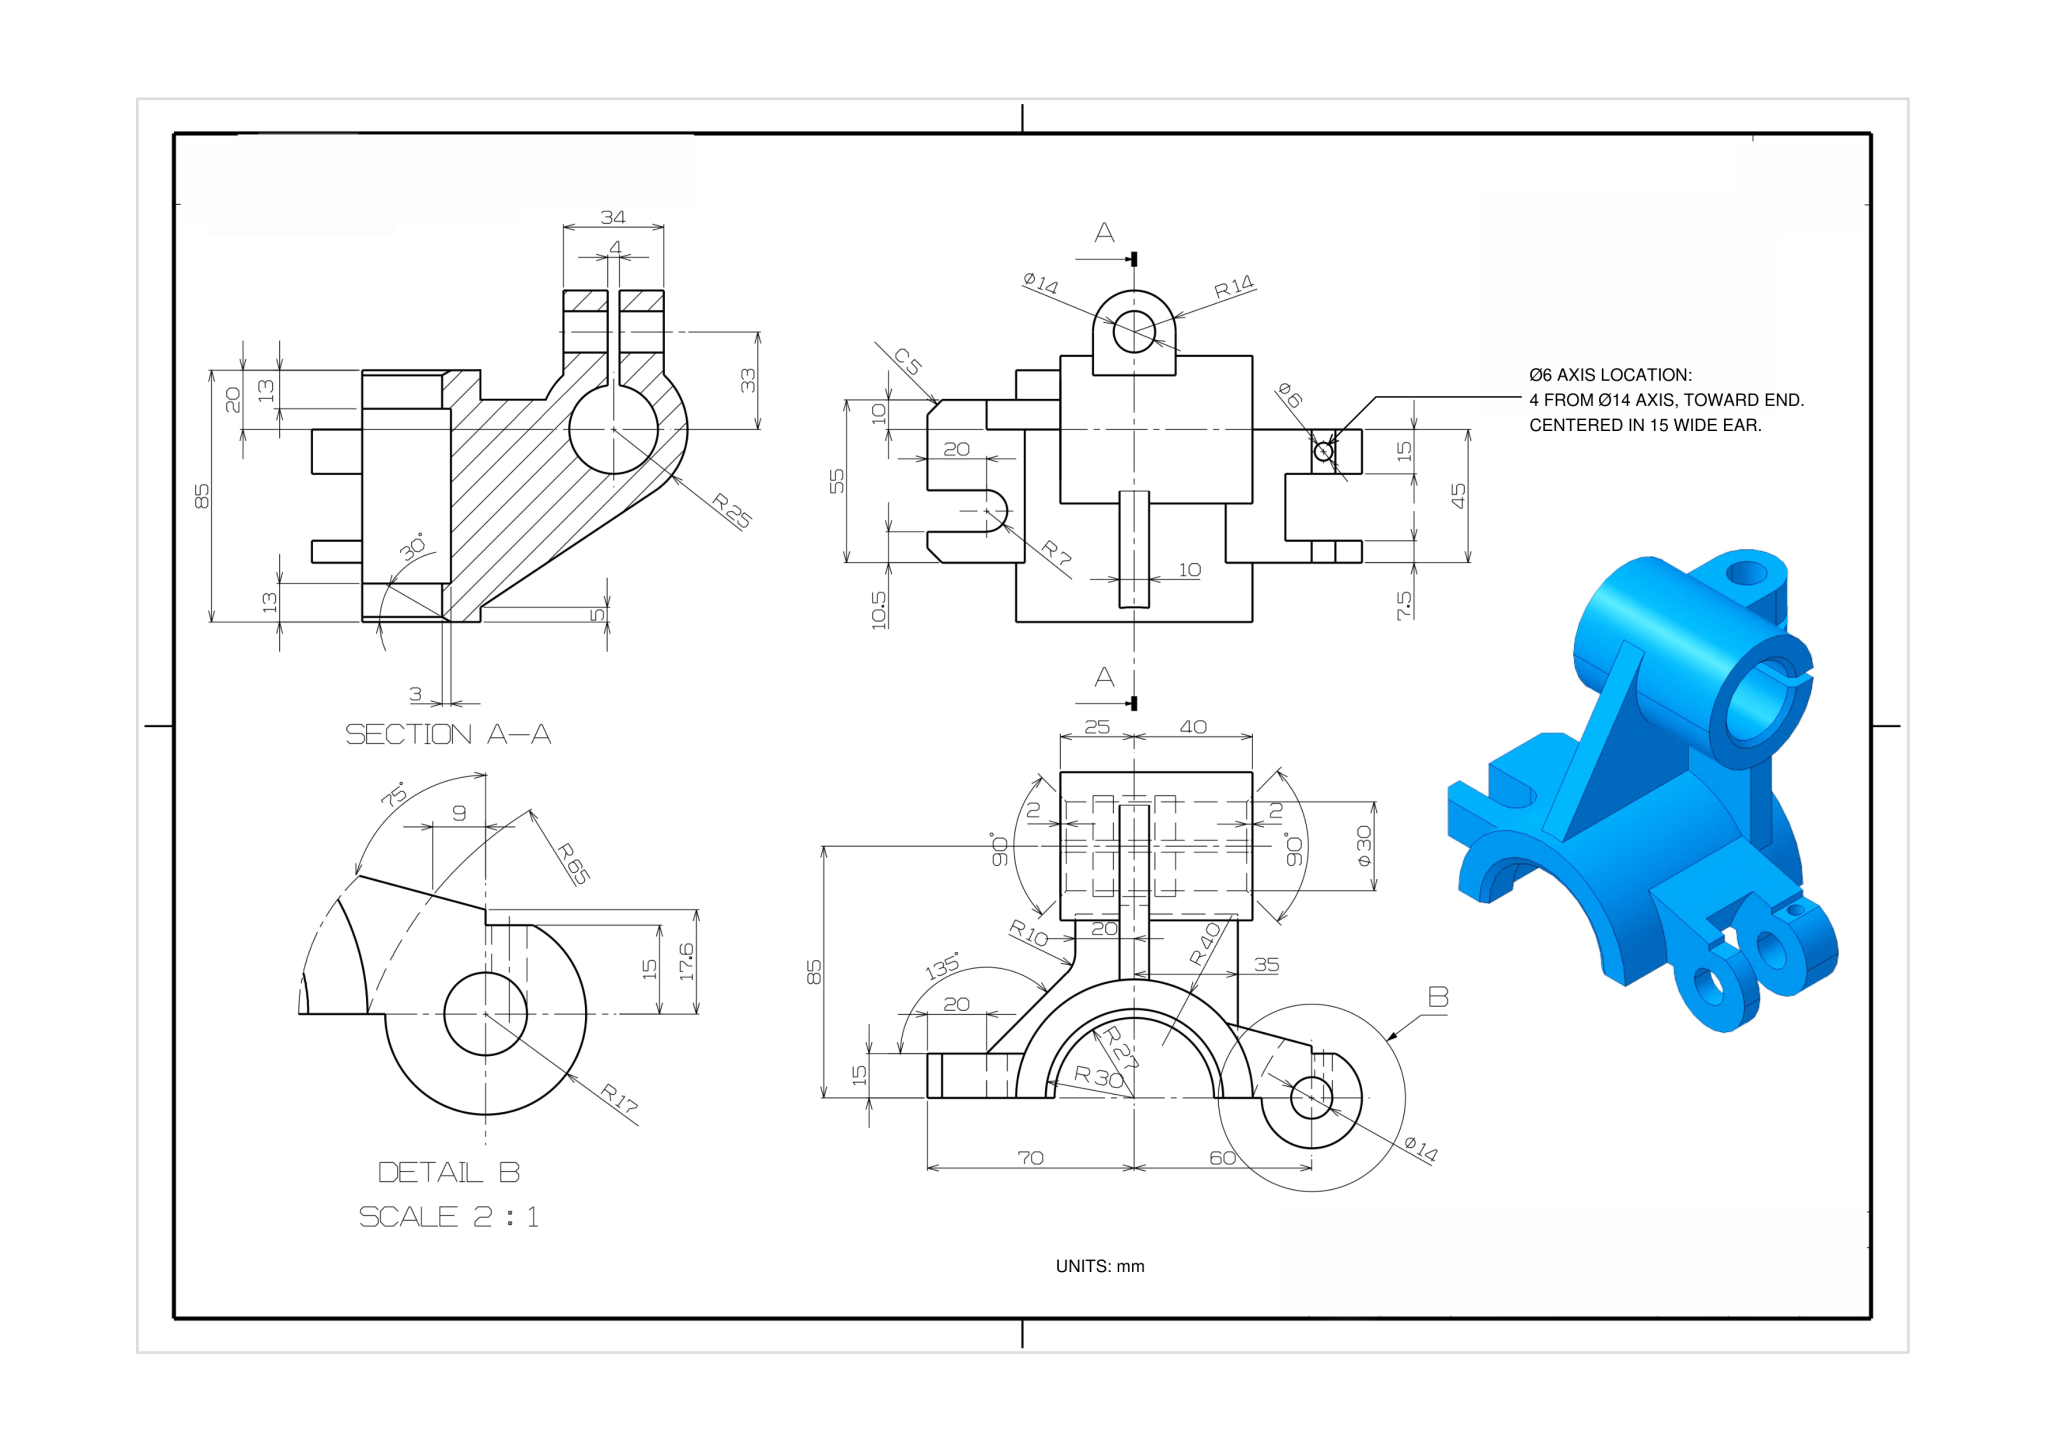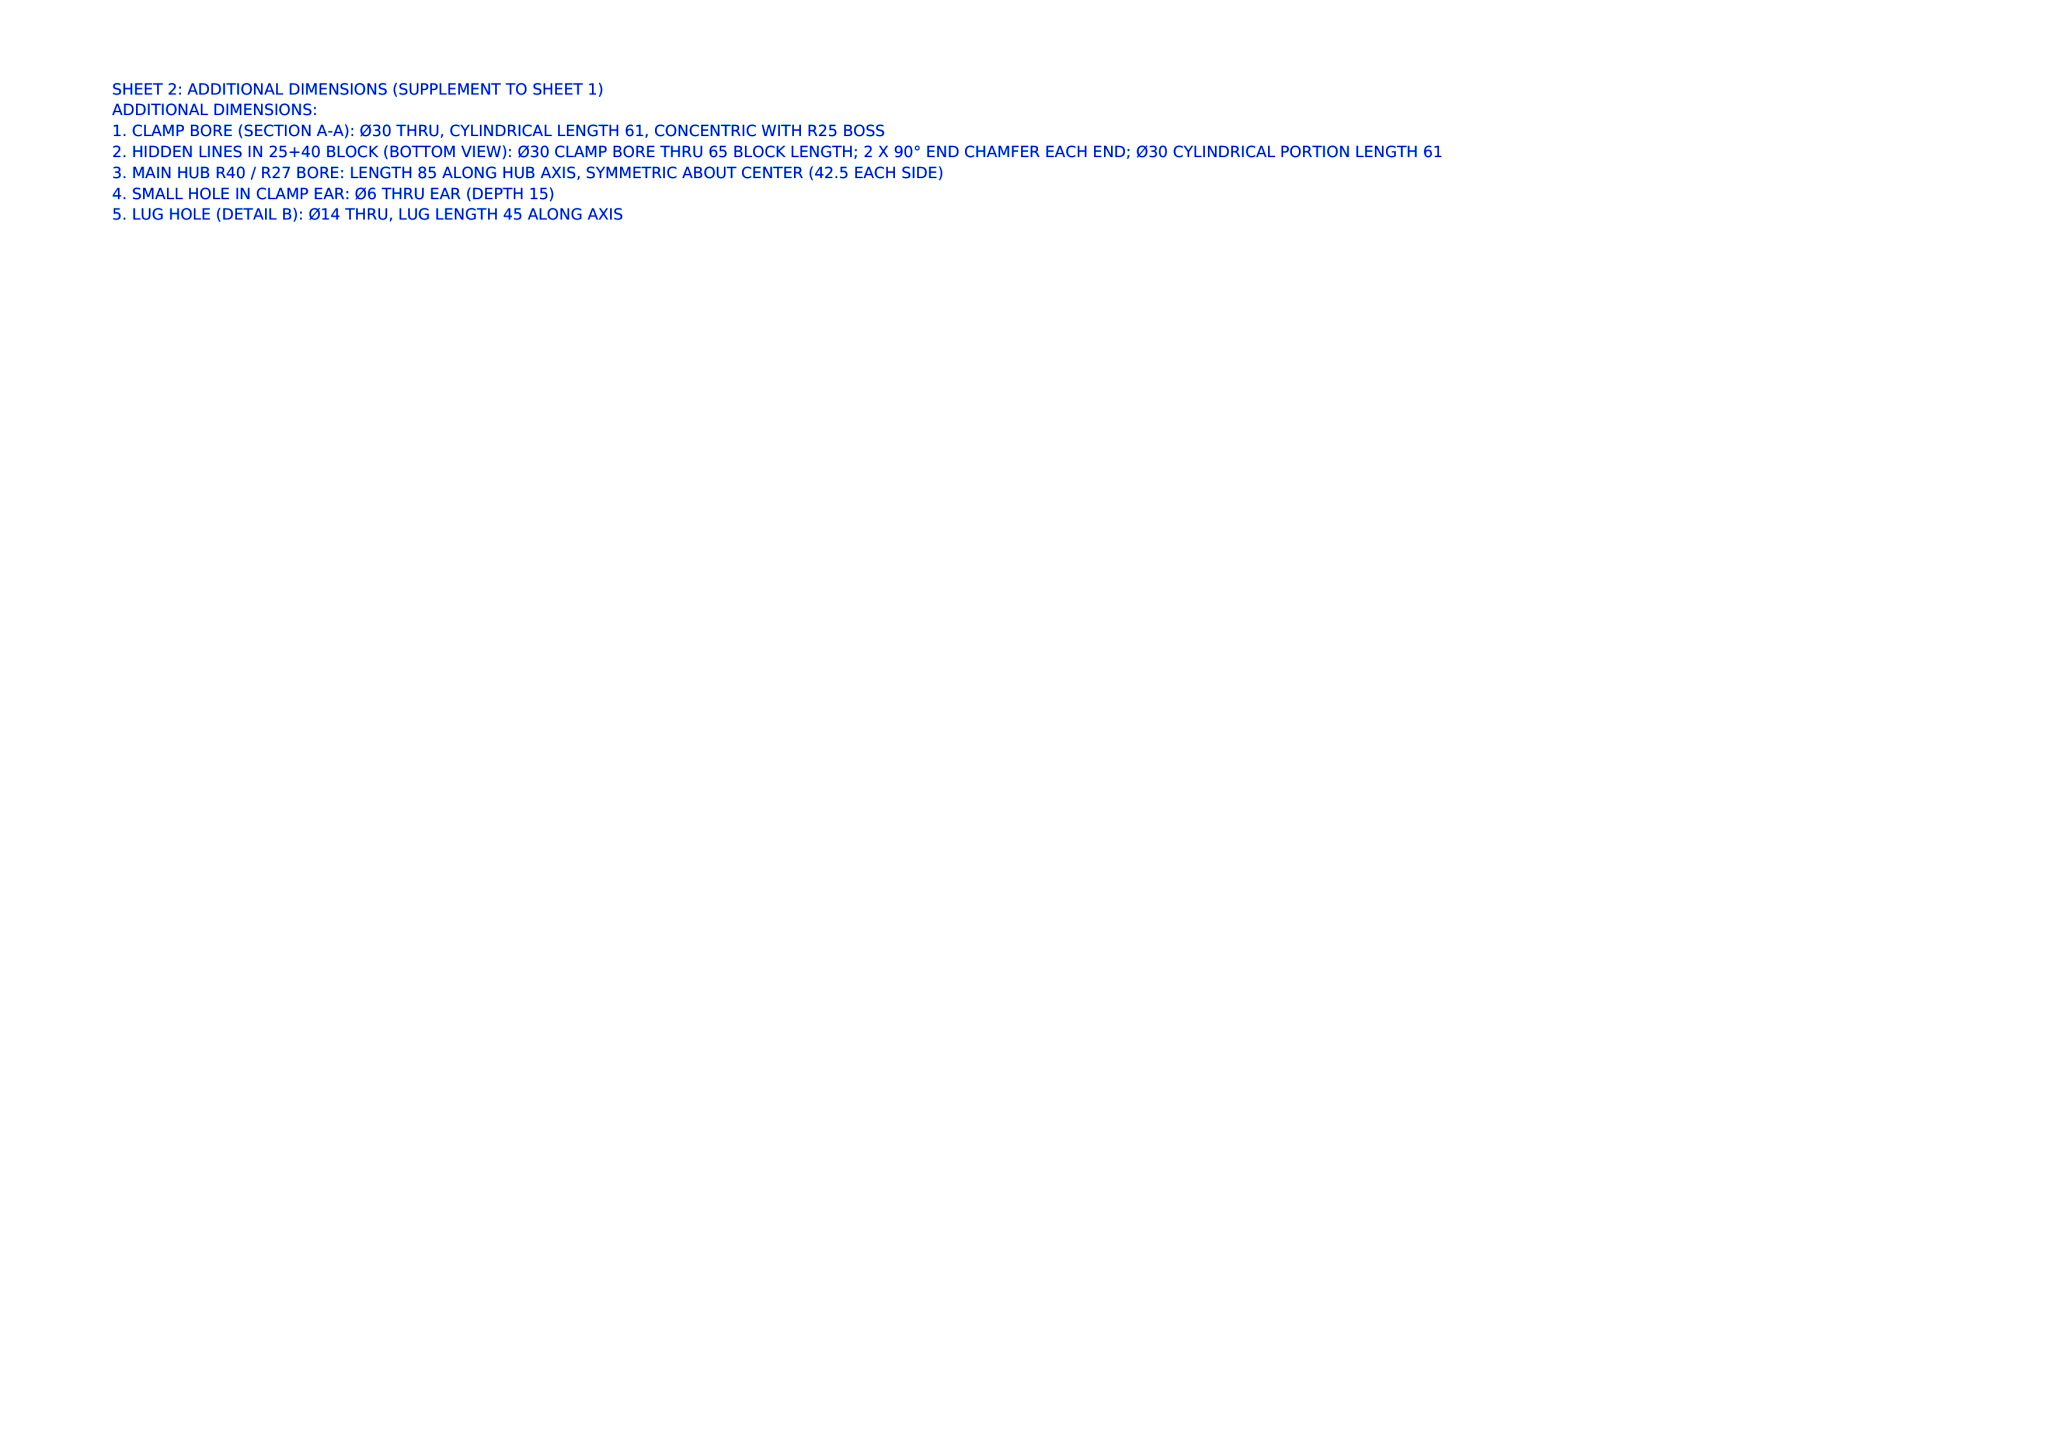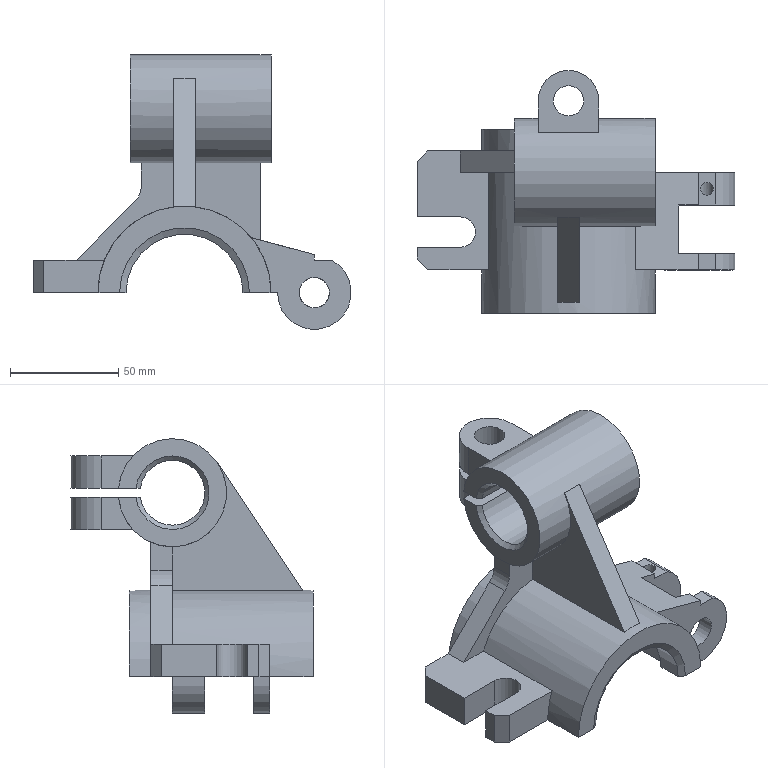Part | NX | mm | 1 solid | 65 faces | box 147 x 112 x 127 mm | volume 269511 mm3 | plane 42 | cylinder 19 | cone 4 | commonest cylinder face diameters 14 x5 80 x2 34 x2 54 x2 28 x2 50 x1 60 x1 130 x1